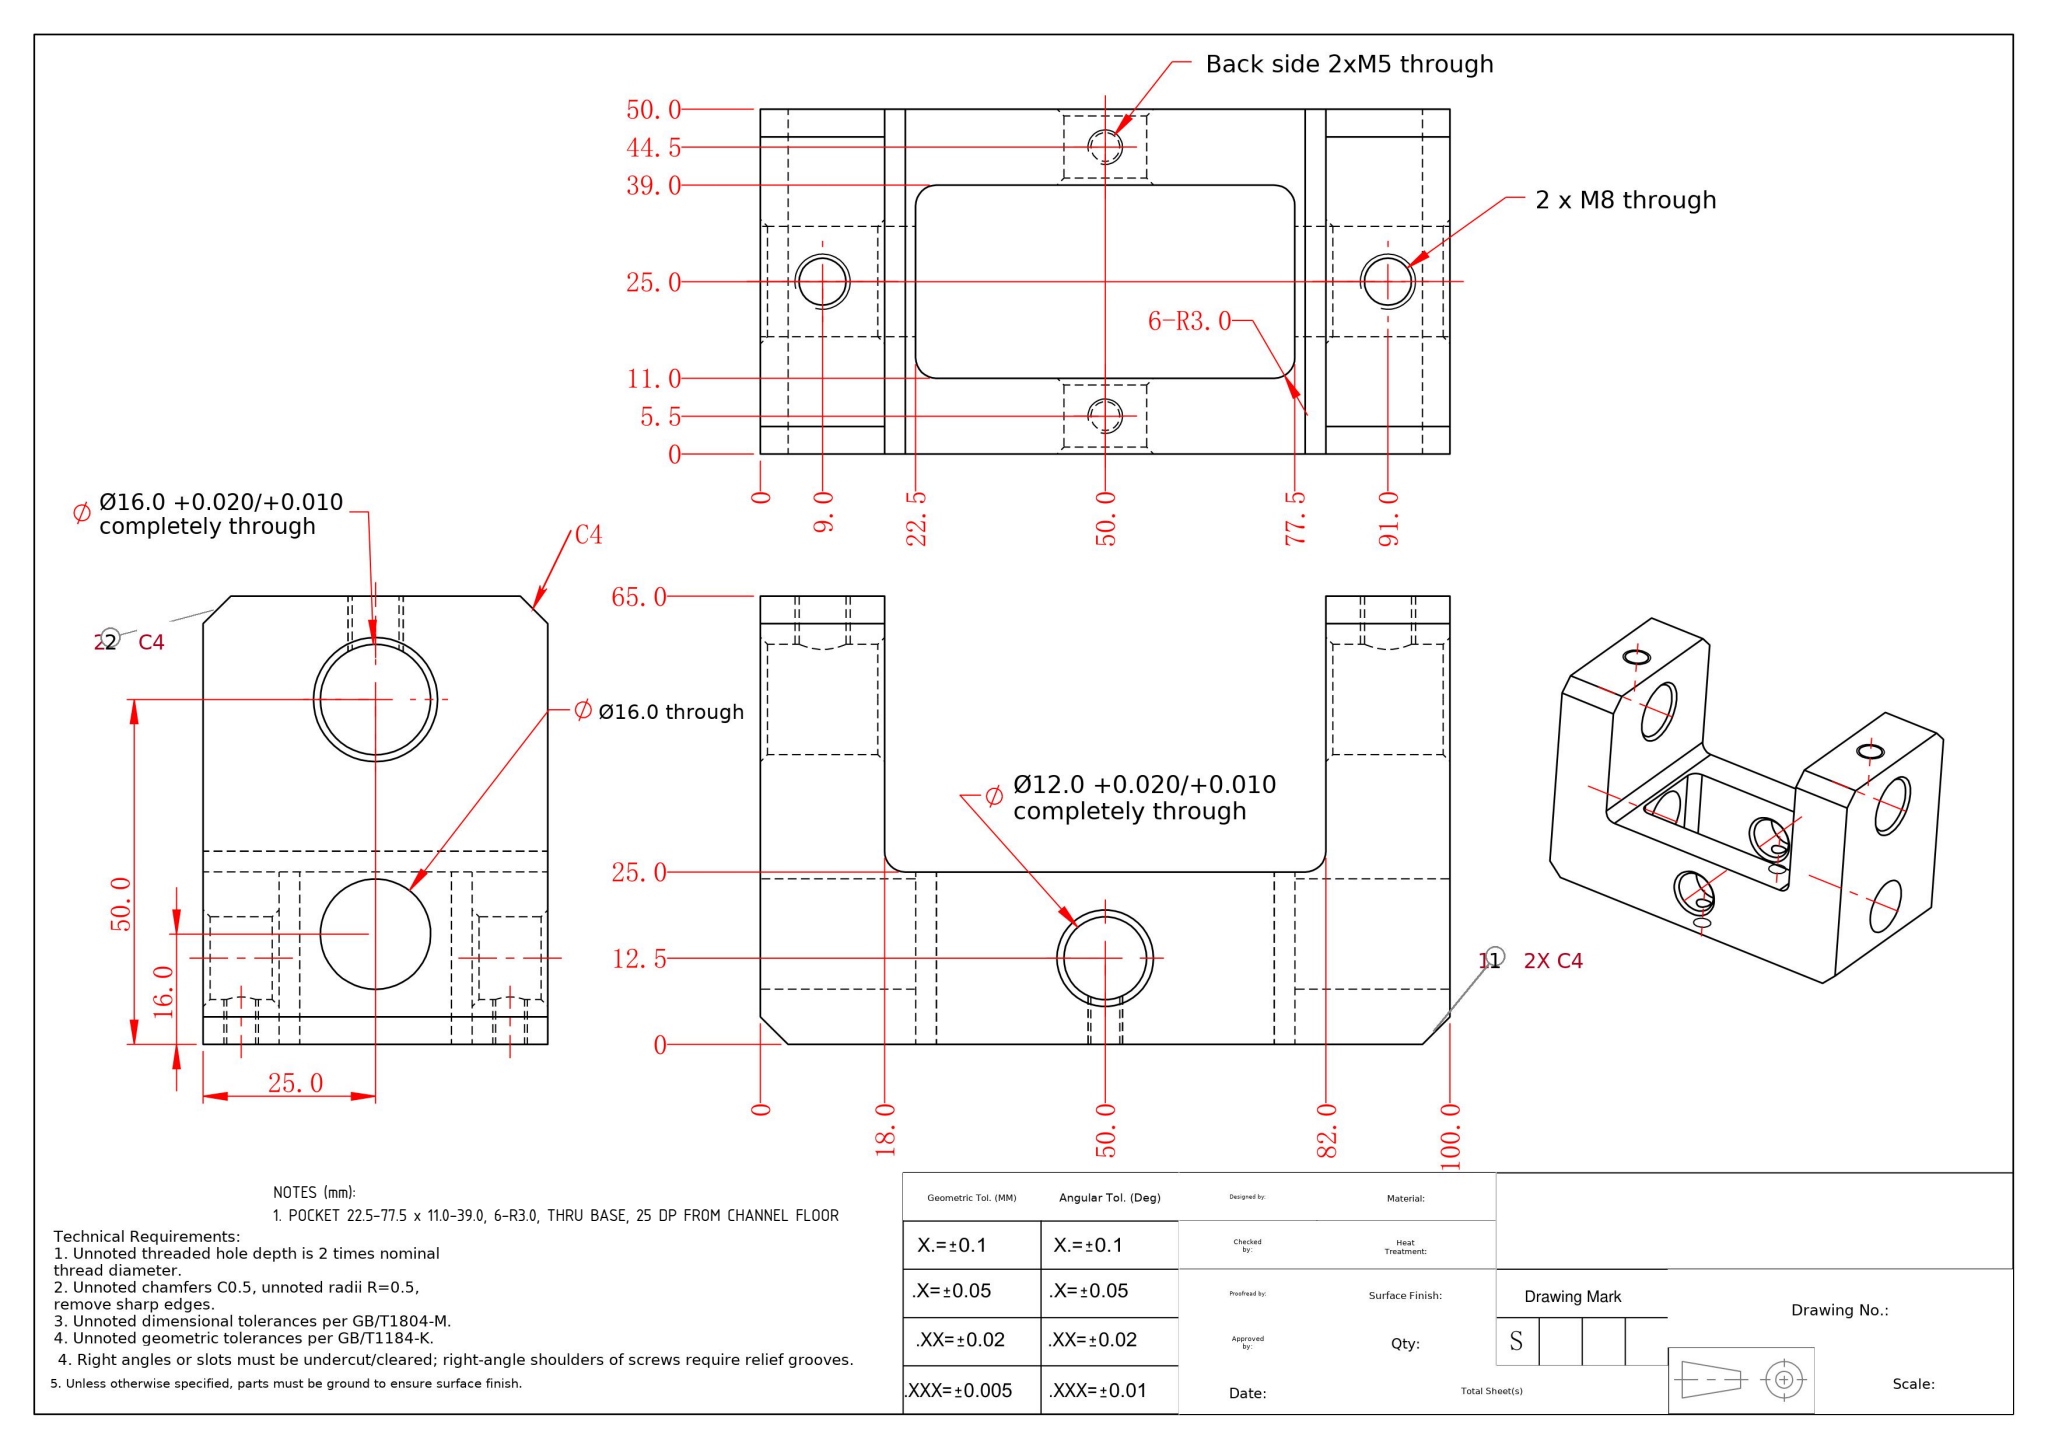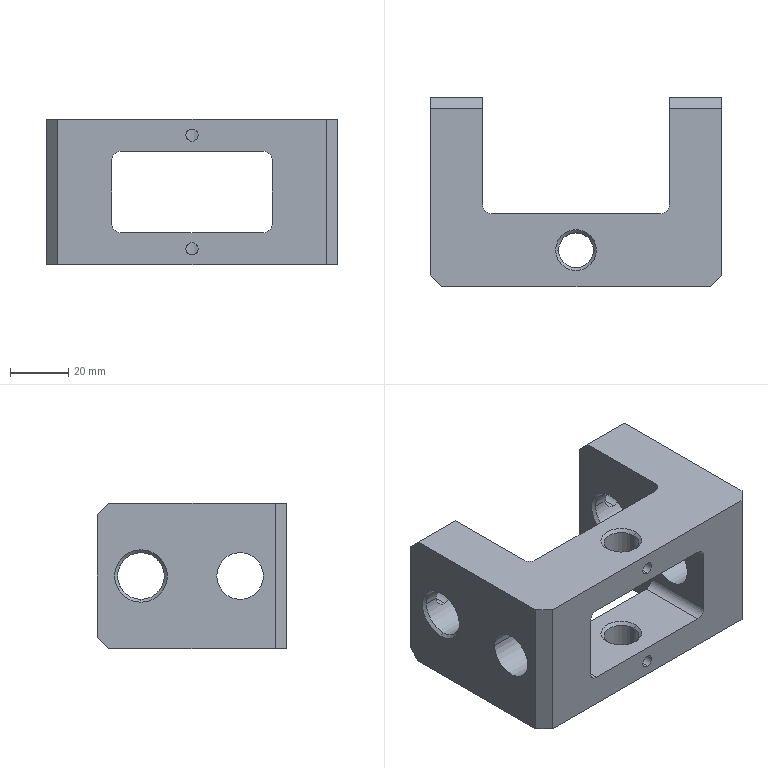Part | SolidWorks | mm | 1 solid | 62 faces | box 100 x 65 x 50 mm | volume 137847 mm3 | cylinder 26 | plane 20 | cone 16 | commonest cylinder face diameters 16 x8 6 x6 4.2 x4 6.8 x4 12 x4
Drawing notes:
POCKET 22.5-77.5 x 11.0-39.0, 6-R3.0, THRU BASE, 25 DP FROM CHANNEL FLOOR | from the solid: Y planes only at 0.0/25.0/65.0; pocket walls x=22.5/77.5, z=11.0/39.0 run from floor y=25.0 to y=0.0; Ø12 hole at (50,12.5) only 9.0+2x1 chamfer long, so base is open z=11-39
build123d program:
from build123d import *

# Parameters (mm, degrees)
BOSS_EXTRUDE1_DEPTH    = 25
SKETCH3_R              = 8
CUT_EXTRUDE1_DEPTH     = 122.861
SKETCH4_W              = 55
SKETCH4_H              = 28
CUT_EXTRUDE2_DEPTH     = 86.732
SKETCH5_R              = 6
CUT_EXTRUDE3_DEPTH     = 97.047
CHAMFER1_SIZE          = 4
FILLET1_R              = 3
M8_TAPPED_HOLE1_REACH  = 87.732
M8_TAPPED_HOLE1_BORE_R = 3.4
M5_TAPPED_HOLE1_REACH  = 87.732
M5_TAPPED_HOLE1_BORE_R = 2.1
CHAMFER2_SIZE          = 1
SKETCH10_R             = 8
CUT_EXTRUDE4_DEPTH     = 122.861


with BuildPart() as part:
    # Sketch1 → Boss-Extrude1 (new, symmetric)
    with BuildSketch(Plane.XY):
        Polygon((-50, 65), (-50, 0), (0, 0), (50, 0), (50, 65), (32, 65), (32, 25), (-32, 25), (-32, 65), align=None)
    extrude(amount=BOSS_EXTRUDE1_DEPTH, both=True)

    # Sketch3 → Cut-Extrude1 (cut, through all)
    with BuildSketch(Plane(origin=(50, 0, 0), x_dir=(0, 0, -1), z_dir=(1, 0, 0))):
        with Locations(Location((0, 50, 0), (0, 0, 90))):
            Circle(SKETCH3_R)
    extrude(amount=-CUT_EXTRUDE1_DEPTH, mode=Mode.SUBTRACT)

    # Sketch4 → Cut-Extrude2 (cut, through all)
    with BuildSketch(Plane.XZ):
        Rectangle(SKETCH4_W, SKETCH4_H)
    extrude(amount=-CUT_EXTRUDE2_DEPTH, mode=Mode.SUBTRACT)

    # Sketch5 → Cut-Extrude3 (cut, through all)
    with BuildSketch(Plane(origin=(0, 0, -25), x_dir=(-1, 0, 0), z_dir=(0, 0, -1))):
        with Locations((0, 12.5)):
            Circle(SKETCH5_R)
    extrude(amount=-CUT_EXTRUDE3_DEPTH, mode=Mode.SUBTRACT)

    # Chamfer1
    chamfer1_edges = [part.edges().sort_by_distance(p)[0] for p in [
        (-41, 65, -25),
        (50, 0, 0),
        (-50, 0, 0),
        (41, 65, 25),
        (-41, 65, 25),
        (41, 65, -25),
    ]]
    chamfer(chamfer1_edges, length=CHAMFER1_SIZE)

    # Fillet1
    fillet1_edges = [part.edges().sort_by_distance(p)[0] for p in [
        (-32, 25, 0),
        (32, 25, 0),
        (27.5, 12.5, 14),
        (27.5, 12.5, -14),
        (-27.5, 12.5, -14),
        (-27.5, 12.5, 14),
    ]]
    fillet(fillet1_edges, radius=FILLET1_R)

    # M8 Tapped Hole1 bore → M8 Tapped Hole1 (cut, up to next)
    with BuildSketch(Plane(origin=(0, 65, 0), x_dir=(1, 0, 0), z_dir=(0, 1, 0)), mode=Mode.PRIVATE) as m8_tapped_hole1_sk1:
        with Locations((41, 0)):
            Circle(M8_TAPPED_HOLE1_BORE_R)
    m8_tapped_hole1_tool1 = extrude(m8_tapped_hole1_sk1.sketch, amount=-M8_TAPPED_HOLE1_REACH, mode=Mode.PRIVATE) & part.part
    # M8 Tapped Hole1 bore → M8 Tapped Hole1 (cut, up to next)
    with BuildSketch(Plane(origin=(0, 65, 0), x_dir=(1, 0, 0), z_dir=(0, 1, 0)), mode=Mode.PRIVATE) as m8_tapped_hole1_sk2:
        with Locations((-41, 0)):
            Circle(M8_TAPPED_HOLE1_BORE_R)
    m8_tapped_hole1_tool2 = extrude(m8_tapped_hole1_sk2.sketch, amount=-M8_TAPPED_HOLE1_REACH, mode=Mode.PRIVATE) & part.part
    add(m8_tapped_hole1_tool1.solids().sort_by_distance((41, 65, 0))[0], mode=Mode.SUBTRACT)
    add(m8_tapped_hole1_tool2.solids().sort_by_distance((-41, 65, 0))[0], mode=Mode.SUBTRACT)

    # M5 Tapped Hole1 bore → M5 Tapped Hole1 (cut, up to next)
    with BuildSketch(Plane(origin=(0, 0, 0), x_dir=(-1, 0, 0), z_dir=(0, -1, 0)), mode=Mode.PRIVATE) as m5_tapped_hole1_sk1:
        with Locations((0, 19.5)):
            Circle(M5_TAPPED_HOLE1_BORE_R)
    m5_tapped_hole1_tool1 = extrude(m5_tapped_hole1_sk1.sketch, amount=-M5_TAPPED_HOLE1_REACH, mode=Mode.PRIVATE) & part.part
    # M5 Tapped Hole1 bore → M5 Tapped Hole1 (cut, up to next)
    with BuildSketch(Plane(origin=(0, 0, 0), x_dir=(-1, 0, 0), z_dir=(0, -1, 0)), mode=Mode.PRIVATE) as m5_tapped_hole1_sk2:
        with Locations((0, -19.5)):
            Circle(M5_TAPPED_HOLE1_BORE_R)
    m5_tapped_hole1_tool2 = extrude(m5_tapped_hole1_sk2.sketch, amount=-M5_TAPPED_HOLE1_REACH, mode=Mode.PRIVATE) & part.part
    add(m5_tapped_hole1_tool1.solids().sort_by_distance((0, 0, -19.5))[0], mode=Mode.SUBTRACT)
    add(m5_tapped_hole1_tool2.solids().sort_by_distance((0, 0, 19.5))[0], mode=Mode.SUBTRACT)

    # Chamfer2
    chamfer2_edges = [part.edges().sort_by_distance(p)[0] for p in [
        (32, 42, 0),
        (-50, 42, 0),
        (-32, 42, 0),
        (50, 42, 0),
        (6, 12.5, -14),
        (6, 12.5, 25),
        (6, 12.5, 14),
        (6, 12.5, -25),
    ]]
    chamfer(chamfer2_edges, length=CHAMFER2_SIZE)

    # Sketch10 → Cut-Extrude4 (cut, through all)
    with BuildSketch(Plane.ZY.offset(50)):
        with Locations(Location((0, 16, 0), (0, 0, 270))):
            Circle(SKETCH10_R)
    extrude(amount=-CUT_EXTRUDE4_DEPTH, mode=Mode.SUBTRACT)


solid = part.part